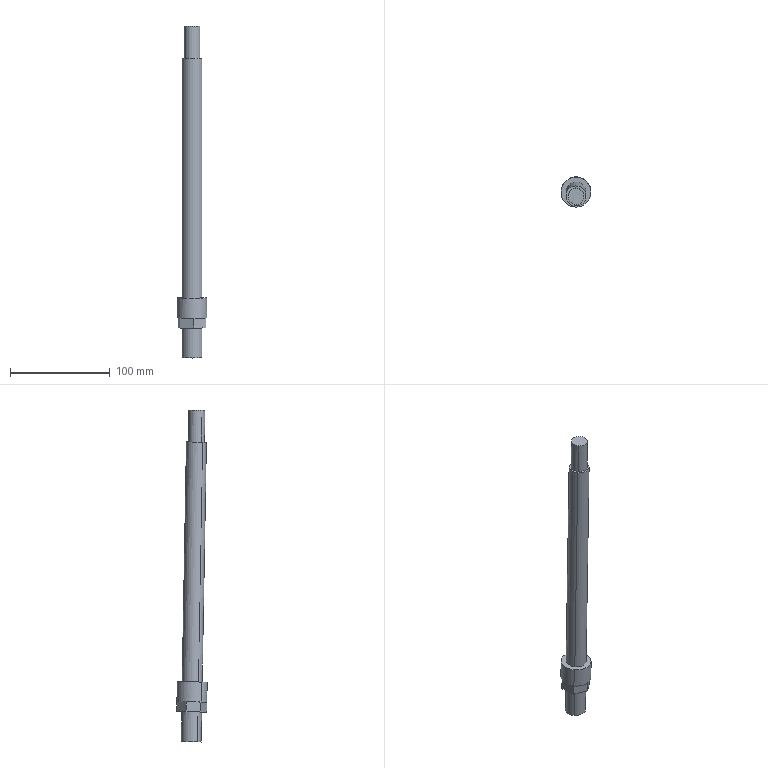Component | SolidWorks | SC63-50CylinderAxis-1 | 1 solid | 25 faces | box 30 x 30.39 x 332.26 mm | volume 111240 mm3 | plane 17 | cylinder 8 | commonest cylinder face diameters 20 x4 16 x2 30 x2
STEP:
#1=CARTESIAN_POINT('',(-1.02,48.421,1.561));
#2=VERTEX_POINT('',#1);
#3=CARTESIAN_POINT('',(-0.3966,48.901,1.569));
#4=VERTEX_POINT('',#3);
#5=CARTESIAN_POINT('',(-0.7085,48.661,1.565));
#6=DIRECTION('',(-0.,-0.01745,0.9998));
#7=DIRECTION('',(-0.7921,-0.6103,-0.01065));
#8=AXIS2_PLACEMENT_3D('',#5,#6,#7);
#9=CIRCLE('',#8,0.3937);
#10=EDGE_CURVE('',#2,#4,#9,.T.);
#11=ORIENTED_EDGE('',*,*,#10,.T.);
#12=CARTESIAN_POINT('',(-0.3966,48.881,2.75));
#13=VERTEX_POINT('',#12);
#14=CARTESIAN_POINT('',(-0.3966,48.673,14.638));
#15=DIRECTION('',(-0.,-0.01745,0.9998));
#16=VECTOR('',#15,39.37);
#17=LINE('',#14,#16);
#18=EDGE_CURVE('',#4,#13,#17,.T.);
#19=ORIENTED_EDGE('',*,*,#18,.T.);
#20=CARTESIAN_POINT('',(-1.02,48.4,2.742));
#21=VERTEX_POINT('',#20);
#22=CARTESIAN_POINT('',(-0.7085,48.641,2.746));
#23=DIRECTION('',(0.,0.01745,-0.9998));
#24=DIRECTION('',(0.7921,0.6103,0.01065));
#25=AXIS2_PLACEMENT_3D('',#22,#23,#24);
#26=CIRCLE('',#25,0.3937);
#27=EDGE_CURVE('',#13,#21,#26,.T.);
#28=ORIENTED_EDGE('',*,*,#27,.T.);
#29=CARTESIAN_POINT('',(-1.02,48.193,14.63));
#30=DIRECTION('',(-0.,-0.01745,0.9998));
#31=VECTOR('',#30,39.37);
#32=LINE('',#29,#31);
#33=EDGE_CURVE('',#2,#21,#32,.T.);
#34=ORIENTED_EDGE('',*,*,#33,.F.);
#35=EDGE_LOOP('',(#11,#19,#28,#34));
#36=FACE_OUTER_BOUND('',#35,.T.);
#37=CARTESIAN_POINT('',(-0.7085,48.433,14.634));
#38=DIRECTION('',(-0.,-0.01745,0.9998));
#39=DIRECTION('',(-0.7921,-0.6103,-0.01065));
#40=AXIS2_PLACEMENT_3D('',#37,#38,#39);
#41=CYLINDRICAL_SURFACE('',#40,0.3937);
#42=ADVANCED_FACE('',(#36),#41,.T.);
#43=CARTESIAN_POINT('',(-0.958,48.263,13.371));
#44=VERTEX_POINT('',#43);
#45=CARTESIAN_POINT('',(-0.459,48.647,13.378));
#46=VERTEX_POINT('',#45);
#47=CARTESIAN_POINT('',(-0.7085,48.455,13.374));
#48=DIRECTION('',(-0.,-0.01745,0.9998));
#49=DIRECTION('',(-0.7921,-0.6103,-0.01065));
#50=AXIS2_PLACEMENT_3D('',#47,#48,#49);
#51=CIRCLE('',#50,0.315);
#52=EDGE_CURVE('',#44,#46,#51,.T.);
#53=ORIENTED_EDGE('',*,*,#52,.T.);
#54=CARTESIAN_POINT('',(-0.459,48.625,14.637));
#55=VERTEX_POINT('',#54);
#56=CARTESIAN_POINT('',(-0.459,48.625,14.637));
#57=DIRECTION('',(-0.,-0.01745,0.9998));
#58=VECTOR('',#57,39.37);
#59=LINE('',#56,#58);
#60=EDGE_CURVE('',#46,#55,#59,.T.);
#61=ORIENTED_EDGE('',*,*,#60,.T.);
#62=CARTESIAN_POINT('',(-0.958,48.241,14.63));
#63=VERTEX_POINT('',#62);
#64=CARTESIAN_POINT('',(-0.7085,48.433,14.634));
#65=DIRECTION('',(-0.,-0.01745,0.9998));
#66=DIRECTION('',(-0.7921,-0.6103,-0.01065));
#67=AXIS2_PLACEMENT_3D('',#64,#65,#66);
#68=CIRCLE('',#67,0.315);
#69=EDGE_CURVE('',#63,#55,#68,.T.);
#70=ORIENTED_EDGE('',*,*,#69,.F.);
#71=CARTESIAN_POINT('',(-0.958,48.241,14.63));
#72=DIRECTION('',(-0.,-0.01745,0.9998));
#73=VECTOR('',#72,39.37);
#74=LINE('',#71,#73);
#75=EDGE_CURVE('',#44,#63,#74,.T.);
#76=ORIENTED_EDGE('',*,*,#75,.F.);
#77=EDGE_LOOP('',(#53,#61,#70,#76));
#78=FACE_OUTER_BOUND('',#77,.T.);
#79=CARTESIAN_POINT('',(-0.7085,48.433,14.634));
#80=DIRECTION('',(-0.,-0.01745,0.9998));
#81=DIRECTION('',(-0.7921,-0.6103,-0.01065));
#82=AXIS2_PLACEMENT_3D('',#79,#80,#81);
#83=CYLINDRICAL_SURFACE('',#82,0.315);
#84=ADVANCED_FACE('',(#78),#83,.T.);
#85=CARTESIAN_POINT('',(-0.3966,48.86,3.931));
#86=VERTEX_POINT('',#85);
#87=CARTESIAN_POINT('',(-1.02,48.38,3.923));
#88=VERTEX_POINT('',#87);
#89=CARTESIAN_POINT('',(-0.7085,48.62,3.927));
#90=DIRECTION('',(0.,0.01745,-0.9998));
#91=DIRECTION('',(0.7921,0.6103,0.01065));
#92=AXIS2_PLACEMENT_3D('',#89,#90,#91);
#93=CIRCLE('',#92,0.3937);
#94=EDGE_CURVE('',#86,#88,#93,.T.);
#95=ORIENTED_EDGE('',*,*,#94,.F.);
#96=CARTESIAN_POINT('',(-0.3966,48.695,13.378));
#97=VERTEX_POINT('',#96);
#98=CARTESIAN_POINT('',(-0.3966,48.673,14.638));
#99=DIRECTION('',(-0.,-0.01745,0.9998));
#100=VECTOR('',#99,39.37);
#101=LINE('',#98,#100);
#102=EDGE_CURVE('',#86,#97,#101,.T.);
#103=ORIENTED_EDGE('',*,*,#102,.T.);
#104=CARTESIAN_POINT('',(-1.02,48.215,13.37));
#105=VERTEX_POINT('',#104);
#106=CARTESIAN_POINT('',(-0.7085,48.455,13.374));
#107=DIRECTION('',(-0.,-0.01745,0.9998));
#108=DIRECTION('',(-0.7921,-0.6103,-0.01065));
#109=AXIS2_PLACEMENT_3D('',#106,#107,#108);
#110=CIRCLE('',#109,0.3937);
#111=EDGE_CURVE('',#105,#97,#110,.T.);
#112=ORIENTED_EDGE('',*,*,#111,.F.);
#113=CARTESIAN_POINT('',(-1.02,48.193,14.63));
#114=DIRECTION('',(-0.,-0.01745,0.9998));
#115=VECTOR('',#114,39.37);
#116=LINE('',#113,#115);
#117=EDGE_CURVE('',#88,#105,#116,.T.);
#118=ORIENTED_EDGE('',*,*,#117,.F.);
#119=EDGE_LOOP('',(#95,#103,#112,#118));
#120=FACE_OUTER_BOUND('',#119,.T.);
#121=CARTESIAN_POINT('',(-0.7085,48.433,14.634));
#122=DIRECTION('',(-0.,-0.01745,0.9998));
#123=DIRECTION('',(-0.7921,-0.6103,-0.01065));
#124=AXIS2_PLACEMENT_3D('',#121,#122,#123);
#125=CYLINDRICAL_SURFACE('',#124,0.3937);
#126=ADVANCED_FACE('',(#120),#125,.T.);
#127=CARTESIAN_POINT('',(-0.2407,48.98,3.933));
#128=VERTEX_POINT('',#127);
#129=CARTESIAN_POINT('',(-1.176,48.26,3.92));
#130=VERTEX_POINT('',#129);
#131=CARTESIAN_POINT('',(-0.7085,48.62,3.927));
#132=DIRECTION('',(0.,0.01745,-0.9998));
#133=DIRECTION('',(0.7921,0.6103,0.01065));
#134=AXIS2_PLACEMENT_3D('',#131,#132,#133);
#135=CIRCLE('',#134,0.5906);
#136=EDGE_CURVE('',#128,#130,#135,.T.);
#137=ORIENTED_EDGE('',*,*,#136,.T.);
#138=CARTESIAN_POINT('',(-1.176,48.273,3.133));
#139=VERTEX_POINT('',#138);
#140=CARTESIAN_POINT('',(-1.176,48.26,3.92));
#141=DIRECTION('',(0.,0.01745,-0.9998));
#142=VECTOR('',#141,39.37);
#143=LINE('',#140,#142);
#144=EDGE_CURVE('',#130,#139,#143,.T.);
#145=ORIENTED_EDGE('',*,*,#144,.T.);
#146=CARTESIAN_POINT('',(-0.6302,48.048,3.129));
#147=VERTEX_POINT('',#146);
#148=CARTESIAN_POINT('',(-0.7085,48.634,3.139));
#149=DIRECTION('',(-0.,-0.01745,0.9998));
#150=DIRECTION('',(0.7921,0.6103,0.01065));
#151=AXIS2_PLACEMENT_3D('',#148,#149,#150);
#152=CIRCLE('',#151,0.5906);
#153=EDGE_CURVE('',#139,#147,#152,.T.);
#154=ORIENTED_EDGE('',*,*,#153,.T.);
#155=CARTESIAN_POINT('',(-0.1625,48.409,3.136));
#156=VERTEX_POINT('',#155);
#157=CARTESIAN_POINT('',(-0.7085,48.634,3.139));
#158=DIRECTION('',(-0.,-0.01745,0.9998));
#159=DIRECTION('',(0.7921,0.6103,0.01065));
#160=AXIS2_PLACEMENT_3D('',#157,#158,#159);
#161=CIRCLE('',#160,0.5906);
#162=EDGE_CURVE('',#147,#156,#161,.T.);
#163=ORIENTED_EDGE('',*,*,#162,.T.);
#164=CARTESIAN_POINT('',(-0.2407,48.994,3.146));
#165=VERTEX_POINT('',#164);
#166=CARTESIAN_POINT('',(-0.7085,48.634,3.139));
#167=DIRECTION('',(-0.,-0.01745,0.9998));
#168=DIRECTION('',(0.7921,0.6103,0.01065));
#169=AXIS2_PLACEMENT_3D('',#166,#167,#168);
#170=CIRCLE('',#169,0.5906);
#171=EDGE_CURVE('',#156,#165,#170,.T.);
#172=ORIENTED_EDGE('',*,*,#171,.T.);
#173=CARTESIAN_POINT('',(-0.2407,48.98,3.933));
#174=DIRECTION('',(0.,0.01745,-0.9998));
#175=VECTOR('',#174,39.37);
#176=LINE('',#173,#175);
#177=EDGE_CURVE('',#128,#165,#176,.T.);
#178=ORIENTED_EDGE('',*,*,#177,.F.);
#179=EDGE_LOOP('',(#137,#145,#154,#163,#172,#178));
#180=FACE_OUTER_BOUND('',#179,.T.);
#181=CARTESIAN_POINT('',(-0.7085,48.62,3.927));
#182=DIRECTION('',(0.,0.01745,-0.9998));
#183=DIRECTION('',(0.7921,0.6103,0.01065));
#184=AXIS2_PLACEMENT_3D('',#181,#182,#183);
#185=CYLINDRICAL_SURFACE('',#184,0.5906);
#186=ADVANCED_FACE('',(#180),#185,.T.);
#187=ORIENTED_EDGE('',*,*,#144,.F.);
#188=CARTESIAN_POINT('',(-0.7085,48.62,3.927));
#189=DIRECTION('',(0.,0.01745,-0.9998));
#190=DIRECTION('',(0.7921,0.6103,0.01065));
#191=AXIS2_PLACEMENT_3D('',#188,#189,#190);
#192=CIRCLE('',#191,0.5906);
#193=EDGE_CURVE('',#130,#128,#192,.T.);
#194=ORIENTED_EDGE('',*,*,#193,.T.);
#195=ORIENTED_EDGE('',*,*,#177,.T.);
#196=CARTESIAN_POINT('',(-0.7868,49.219,3.15));
#197=VERTEX_POINT('',#196);
#198=CARTESIAN_POINT('',(-0.7085,48.634,3.139));
#199=DIRECTION('',(-0.,-0.01745,0.9998));
#200=DIRECTION('',(0.7921,0.6103,0.01065));
#201=AXIS2_PLACEMENT_3D('',#198,#199,#200);
#202=CIRCLE('',#201,0.5906);
#203=EDGE_CURVE('',#165,#197,#202,.T.);
#204=ORIENTED_EDGE('',*,*,#203,.T.);
#205=CARTESIAN_POINT('',(-1.255,48.859,3.143));
#206=VERTEX_POINT('',#205);
#207=CARTESIAN_POINT('',(-0.7085,48.634,3.139));
#208=DIRECTION('',(-0.,-0.01745,0.9998));
#209=DIRECTION('',(0.7921,0.6103,0.01065));
#210=AXIS2_PLACEMENT_3D('',#207,#208,#209);
#211=CIRCLE('',#210,0.5906);
#212=EDGE_CURVE('',#197,#206,#211,.T.);
#213=ORIENTED_EDGE('',*,*,#212,.T.);
#214=CARTESIAN_POINT('',(-0.7085,48.634,3.139));
#215=DIRECTION('',(-0.,-0.01745,0.9998));
#216=DIRECTION('',(0.7921,0.6103,0.01065));
#217=AXIS2_PLACEMENT_3D('',#214,#215,#216);
#218=CIRCLE('',#217,0.5906);
#219=EDGE_CURVE('',#206,#139,#218,.T.);
#220=ORIENTED_EDGE('',*,*,#219,.T.);
#221=EDGE_LOOP('',(#187,#194,#195,#204,#213,#220));
#222=FACE_OUTER_BOUND('',#221,.T.);
#223=CARTESIAN_POINT('',(-0.7085,48.62,3.927));
#224=DIRECTION('',(0.,0.01745,-0.9998));
#225=DIRECTION('',(0.7921,0.6103,0.01065));
#226=AXIS2_PLACEMENT_3D('',#223,#224,#225);
#227=CYLINDRICAL_SURFACE('',#226,0.5906);
#228=ADVANCED_FACE('',(#222),#227,.T.);
#229=ORIENTED_EDGE('',*,*,#102,.F.);
#230=CARTESIAN_POINT('',(-0.7085,48.62,3.927));
#231=DIRECTION('',(0.,0.01745,-0.9998));
#232=DIRECTION('',(0.7921,0.6103,0.01065));
#233=AXIS2_PLACEMENT_3D('',#230,#231,#232);
#234=CIRCLE('',#233,0.3937);
#235=EDGE_CURVE('',#88,#86,#234,.T.);
#236=ORIENTED_EDGE('',*,*,#235,.F.);
#237=ORIENTED_EDGE('',*,*,#117,.T.);
#238=CARTESIAN_POINT('',(-0.7085,48.455,13.374));
#239=DIRECTION('',(-0.,-0.01745,0.9998));
#240=DIRECTION('',(-0.7921,-0.6103,-0.01065));
#241=AXIS2_PLACEMENT_3D('',#238,#239,#240);
#242=CIRCLE('',#241,0.3937);
#243=EDGE_CURVE('',#97,#105,#242,.T.);
#244=ORIENTED_EDGE('',*,*,#243,.F.);
#245=EDGE_LOOP('',(#229,#236,#237,#244));
#246=FACE_OUTER_BOUND('',#245,.T.);
#247=CARTESIAN_POINT('',(-0.7085,48.433,14.634));
#248=DIRECTION('',(-0.,-0.01745,0.9998));
#249=DIRECTION('',(-0.7921,-0.6103,-0.01065));
#250=AXIS2_PLACEMENT_3D('',#247,#248,#249);
#251=CYLINDRICAL_SURFACE('',#250,0.3937);
#252=ADVANCED_FACE('',(#246),#251,.T.);
#253=ORIENTED_EDGE('',*,*,#69,.T.);
#254=CARTESIAN_POINT('',(-0.7085,48.433,14.634));
#255=DIRECTION('',(-0.,-0.01745,0.9998));
#256=DIRECTION('',(-0.7921,-0.6103,-0.01065));
#257=AXIS2_PLACEMENT_3D('',#254,#255,#256);
#258=CIRCLE('',#257,0.315);
#259=EDGE_CURVE('',#55,#63,#258,.T.);
#260=ORIENTED_EDGE('',*,*,#259,.T.);
#261=EDGE_LOOP('',(#253,#260));
#262=FACE_OUTER_BOUND('',#261,.T.);
#263=CARTESIAN_POINT('',(-0.7085,48.433,14.634));
#264=DIRECTION('',(0.,0.01745,-0.9998));
#265=DIRECTION('',(0.7921,0.6103,0.01065));
#266=AXIS2_PLACEMENT_3D('',#263,#264,#265);
#267=PLANE('',#266);
#268=ADVANCED_FACE('',(#262),#267,.F.);
#269=ORIENTED_EDGE('',*,*,#60,.F.);
#270=CARTESIAN_POINT('',(-0.7085,48.455,13.374));
#271=DIRECTION('',(-0.,-0.01745,0.9998));
#272=DIRECTION('',(-0.7921,-0.6103,-0.01065));
#273=AXIS2_PLACEMENT_3D('',#270,#271,#272);
#274=CIRCLE('',#273,0.315);
#275=EDGE_CURVE('',#46,#44,#274,.T.);
#276=ORIENTED_EDGE('',*,*,#275,.T.);
#277=ORIENTED_EDGE('',*,*,#75,.T.);
#278=ORIENTED_EDGE('',*,*,#259,.F.);
#279=EDGE_LOOP('',(#269,#276,#277,#278));
#280=FACE_OUTER_BOUND('',#279,.T.);
#281=CARTESIAN_POINT('',(-0.7085,48.433,14.634));
#282=DIRECTION('',(-0.,-0.01745,0.9998));
#283=DIRECTION('',(-0.7921,-0.6103,-0.01065));
#284=AXIS2_PLACEMENT_3D('',#281,#282,#283);
#285=CYLINDRICAL_SURFACE('',#284,0.315);
#286=ADVANCED_FACE('',(#280),#285,.T.);
#287=ORIENTED_EDGE('',*,*,#52,.F.);
#288=ORIENTED_EDGE('',*,*,#275,.F.);
#289=EDGE_LOOP('',(#287,#288));
#290=FACE_BOUND('',#289,.T.);
#291=ORIENTED_EDGE('',*,*,#111,.T.);
#292=ORIENTED_EDGE('',*,*,#243,.T.);
#293=EDGE_LOOP('',(#291,#292));
#294=FACE_OUTER_BOUND('',#293,.T.);
#295=CARTESIAN_POINT('',(-0.5163,48.206,13.37));
#296=DIRECTION('',(0.,0.01745,-0.9998));
#297=DIRECTION('',(0.7921,0.6103,0.01065));
#298=AXIS2_PLACEMENT_3D('',#295,#296,#297);
#299=PLANE('',#298);
#300=ADVANCED_FACE('',(#290,#294),#299,.F.);
#301=ORIENTED_EDGE('',*,*,#235,.T.);
#302=ORIENTED_EDGE('',*,*,#94,.T.);
#303=EDGE_LOOP('',(#301,#302));
#304=FACE_BOUND('',#303,.T.);
#305=ORIENTED_EDGE('',*,*,#136,.F.);
#306=ORIENTED_EDGE('',*,*,#193,.F.);
#307=EDGE_LOOP('',(#305,#306));
#308=FACE_OUTER_BOUND('',#307,.T.);
#309=CARTESIAN_POINT('',(-0.7085,48.62,3.927));
#310=DIRECTION('',(0.,0.01745,-0.9998));
#311=DIRECTION('',(0.7921,0.6103,0.01065));
#312=AXIS2_PLACEMENT_3D('',#309,#310,#311);
#313=PLANE('',#312);
#314=ADVANCED_FACE('',(#304,#308),#313,.F.);
#315=CARTESIAN_POINT('',(-0.7868,49.219,3.15));
#316=DIRECTION('',(0.9246,-0.3808,-0.006646));
#317=VECTOR('',#316,39.37);
#318=LINE('',#315,#317);
#319=EDGE_CURVE('',#197,#165,#318,.T.);
#320=ORIENTED_EDGE('',*,*,#319,.F.);
#321=ORIENTED_EDGE('',*,*,#203,.F.);
#322=EDGE_LOOP('',(#320,#321));
#323=FACE_OUTER_BOUND('',#322,.T.);
#324=CARTESIAN_POINT('',(-0.7085,48.634,3.139));
#325=DIRECTION('',(0.,0.01745,-0.9998));
#326=DIRECTION('',(0.7921,0.6103,0.01065));
#327=AXIS2_PLACEMENT_3D('',#324,#325,#326);
#328=PLANE('',#327);
#329=ADVANCED_FACE('',(#323),#328,.T.);
#330=CARTESIAN_POINT('',(-1.255,48.859,3.143));
#331=DIRECTION('',(0.7921,0.6103,0.01065));
#332=VECTOR('',#331,39.37);
#333=LINE('',#330,#332);
#334=EDGE_CURVE('',#206,#197,#333,.T.);
#335=ORIENTED_EDGE('',*,*,#334,.F.);
#336=ORIENTED_EDGE('',*,*,#212,.F.);
#337=EDGE_LOOP('',(#335,#336));
#338=FACE_OUTER_BOUND('',#337,.T.);
#339=CARTESIAN_POINT('',(-0.7085,48.634,3.139));
#340=DIRECTION('',(0.,0.01745,-0.9998));
#341=DIRECTION('',(0.7921,0.6103,0.01065));
#342=AXIS2_PLACEMENT_3D('',#339,#340,#341);
#343=PLANE('',#342);
#344=ADVANCED_FACE('',(#338),#343,.T.);
#345=CARTESIAN_POINT('',(-1.176,48.273,3.133));
#346=DIRECTION('',(-0.1325,0.991,0.0173));
#347=VECTOR('',#346,39.37);
#348=LINE('',#345,#347);
#349=EDGE_CURVE('',#139,#206,#348,.T.);
#350=ORIENTED_EDGE('',*,*,#349,.F.);
#351=ORIENTED_EDGE('',*,*,#219,.F.);
#352=EDGE_LOOP('',(#350,#351));
#353=FACE_OUTER_BOUND('',#352,.T.);
#354=CARTESIAN_POINT('',(-0.7085,48.634,3.139));
#355=DIRECTION('',(0.,0.01745,-0.9998));
#356=DIRECTION('',(0.7921,0.6103,0.01065));
#357=AXIS2_PLACEMENT_3D('',#354,#355,#356);
#358=PLANE('',#357);
#359=ADVANCED_FACE('',(#353),#358,.T.);
#360=CARTESIAN_POINT('',(-0.6302,48.048,3.129));
#361=DIRECTION('',(-0.9246,0.3808,0.006646));
#362=VECTOR('',#361,39.37);
#363=LINE('',#360,#362);
#364=EDGE_CURVE('',#147,#139,#363,.T.);
#365=ORIENTED_EDGE('',*,*,#364,.F.);
#366=ORIENTED_EDGE('',*,*,#153,.F.);
#367=EDGE_LOOP('',(#365,#366));
#368=FACE_OUTER_BOUND('',#367,.T.);
#369=CARTESIAN_POINT('',(-0.7085,48.634,3.139));
#370=DIRECTION('',(0.,0.01745,-0.9998));
#371=DIRECTION('',(0.7921,0.6103,0.01065));
#372=AXIS2_PLACEMENT_3D('',#369,#370,#371);
#373=PLANE('',#372);
#374=ADVANCED_FACE('',(#368),#373,.T.);
#375=CARTESIAN_POINT('',(-0.1625,48.409,3.136));
#376=DIRECTION('',(-0.7921,-0.6103,-0.01065));
#377=VECTOR('',#376,39.37);
#378=LINE('',#375,#377);
#379=EDGE_CURVE('',#156,#147,#378,.T.);
#380=ORIENTED_EDGE('',*,*,#379,.F.);
#381=ORIENTED_EDGE('',*,*,#162,.F.);
#382=EDGE_LOOP('',(#380,#381));
#383=FACE_OUTER_BOUND('',#382,.T.);
#384=CARTESIAN_POINT('',(-0.7085,48.634,3.139));
#385=DIRECTION('',(0.,0.01745,-0.9998));
#386=DIRECTION('',(0.7921,0.6103,0.01065));
#387=AXIS2_PLACEMENT_3D('',#384,#385,#386);
#388=PLANE('',#387);
#389=ADVANCED_FACE('',(#383),#388,.T.);
#390=CARTESIAN_POINT('',(-0.2407,48.994,3.146));
#391=DIRECTION('',(0.1325,-0.991,-0.0173));
#392=VECTOR('',#391,39.37);
#393=LINE('',#390,#392);
#394=EDGE_CURVE('',#165,#156,#393,.T.);
#395=ORIENTED_EDGE('',*,*,#394,.F.);
#396=ORIENTED_EDGE('',*,*,#171,.F.);
#397=EDGE_LOOP('',(#395,#396));
#398=FACE_OUTER_BOUND('',#397,.T.);
#399=CARTESIAN_POINT('',(-0.7085,48.634,3.139));
#400=DIRECTION('',(0.,0.01745,-0.9998));
#401=DIRECTION('',(0.7921,0.6103,0.01065));
#402=AXIS2_PLACEMENT_3D('',#399,#400,#401);
#403=PLANE('',#402);
#404=ADVANCED_FACE('',(#398),#403,.T.);
#405=CARTESIAN_POINT('',(-0.7868,49.226,2.756));
#406=VERTEX_POINT('',#405);
#407=CARTESIAN_POINT('',(-0.2407,49.001,2.752));
#408=VERTEX_POINT('',#407);
#409=CARTESIAN_POINT('',(-0.7868,49.226,2.756));
#410=DIRECTION('',(0.9246,-0.3808,-0.006646));
#411=VECTOR('',#410,39.37);
#412=LINE('',#409,#411);
#413=EDGE_CURVE('',#406,#408,#412,.T.);
#414=ORIENTED_EDGE('',*,*,#413,.F.);
#415=CARTESIAN_POINT('',(-0.7868,49.219,3.15));
#416=DIRECTION('',(0.,0.01745,-0.9998));
#417=VECTOR('',#416,39.37);
#418=LINE('',#415,#417);
#419=EDGE_CURVE('',#197,#406,#418,.T.);
#420=ORIENTED_EDGE('',*,*,#419,.F.);
#421=ORIENTED_EDGE('',*,*,#319,.T.);
#422=CARTESIAN_POINT('',(-0.2407,48.994,3.146));
#423=DIRECTION('',(0.,0.01745,-0.9998));
#424=VECTOR('',#423,39.37);
#425=LINE('',#422,#424);
#426=EDGE_CURVE('',#165,#408,#425,.T.);
#427=ORIENTED_EDGE('',*,*,#426,.T.);
#428=EDGE_LOOP('',(#414,#420,#421,#427));
#429=FACE_OUTER_BOUND('',#428,.T.);
#430=CARTESIAN_POINT('',(-0.7868,49.219,3.15));
#431=DIRECTION('',(0.3808,0.9245,0.01614));
#432=DIRECTION('',(0.9246,-0.3808,-0.006646));
#433=AXIS2_PLACEMENT_3D('',#430,#431,#432);
#434=PLANE('',#433);
#435=ADVANCED_FACE('',(#429),#434,.T.);
#436=CARTESIAN_POINT('',(-1.255,48.865,2.75));
#437=VERTEX_POINT('',#436);
#438=CARTESIAN_POINT('',(-1.255,48.865,2.75));
#439=DIRECTION('',(0.7921,0.6103,0.01065));
#440=VECTOR('',#439,39.37);
#441=LINE('',#438,#440);
#442=EDGE_CURVE('',#437,#406,#441,.T.);
#443=ORIENTED_EDGE('',*,*,#442,.F.);
#444=CARTESIAN_POINT('',(-1.255,48.859,3.143));
#445=DIRECTION('',(0.,0.01745,-0.9998));
#446=VECTOR('',#445,39.37);
#447=LINE('',#444,#446);
#448=EDGE_CURVE('',#206,#437,#447,.T.);
#449=ORIENTED_EDGE('',*,*,#448,.F.);
#450=ORIENTED_EDGE('',*,*,#334,.T.);
#451=ORIENTED_EDGE('',*,*,#419,.T.);
#452=EDGE_LOOP('',(#443,#449,#450,#451));
#453=FACE_OUTER_BOUND('',#452,.T.);
#454=CARTESIAN_POINT('',(-1.255,48.859,3.143));
#455=DIRECTION('',(-0.6104,0.792,0.01382));
#456=DIRECTION('',(0.7921,0.6103,0.01065));
#457=AXIS2_PLACEMENT_3D('',#454,#455,#456);
#458=PLANE('',#457);
#459=ADVANCED_FACE('',(#453),#458,.T.);
#460=CARTESIAN_POINT('',(-1.176,48.28,2.74));
#461=VERTEX_POINT('',#460);
#462=CARTESIAN_POINT('',(-1.176,48.28,2.74));
#463=DIRECTION('',(-0.1325,0.991,0.0173));
#464=VECTOR('',#463,39.37);
#465=LINE('',#462,#464);
#466=EDGE_CURVE('',#461,#437,#465,.T.);
#467=ORIENTED_EDGE('',*,*,#466,.F.);
#468=CARTESIAN_POINT('',(-1.176,48.273,3.133));
#469=DIRECTION('',(0.,0.01745,-0.9998));
#470=VECTOR('',#469,39.37);
#471=LINE('',#468,#470);
#472=EDGE_CURVE('',#139,#461,#471,.T.);
#473=ORIENTED_EDGE('',*,*,#472,.F.);
#474=ORIENTED_EDGE('',*,*,#349,.T.);
#475=ORIENTED_EDGE('',*,*,#448,.T.);
#476=EDGE_LOOP('',(#467,#473,#474,#475));
#477=FACE_OUTER_BOUND('',#476,.T.);
#478=CARTESIAN_POINT('',(-1.176,48.273,3.133));
#479=DIRECTION('',(-0.9912,-0.1325,-0.002313));
#480=DIRECTION('',(-0.1325,0.991,0.0173));
#481=AXIS2_PLACEMENT_3D('',#478,#479,#480);
#482=PLANE('',#481);
#483=ADVANCED_FACE('',(#477),#482,.T.);
#484=CARTESIAN_POINT('',(-0.6302,48.055,2.736));
#485=VERTEX_POINT('',#484);
#486=CARTESIAN_POINT('',(-0.6302,48.055,2.736));
#487=DIRECTION('',(-0.9246,0.3808,0.006646));
#488=VECTOR('',#487,39.37);
#489=LINE('',#486,#488);
#490=EDGE_CURVE('',#485,#461,#489,.T.);
#491=ORIENTED_EDGE('',*,*,#490,.F.);
#492=CARTESIAN_POINT('',(-0.6302,48.048,3.129));
#493=DIRECTION('',(0.,0.01745,-0.9998));
#494=VECTOR('',#493,39.37);
#495=LINE('',#492,#494);
#496=EDGE_CURVE('',#147,#485,#495,.T.);
#497=ORIENTED_EDGE('',*,*,#496,.F.);
#498=ORIENTED_EDGE('',*,*,#364,.T.);
#499=ORIENTED_EDGE('',*,*,#472,.T.);
#500=EDGE_LOOP('',(#491,#497,#498,#499));
#501=FACE_OUTER_BOUND('',#500,.T.);
#502=CARTESIAN_POINT('',(-0.6302,48.048,3.129));
#503=DIRECTION('',(-0.3808,-0.9245,-0.01614));
#504=DIRECTION('',(-0.9246,0.3808,0.006646));
#505=AXIS2_PLACEMENT_3D('',#502,#503,#504);
#506=PLANE('',#505);
#507=ADVANCED_FACE('',(#501),#506,.T.);
#508=CARTESIAN_POINT('',(-0.1625,48.416,2.742));
#509=VERTEX_POINT('',#508);
#510=CARTESIAN_POINT('',(-0.1625,48.416,2.742));
#511=DIRECTION('',(-0.7921,-0.6103,-0.01065));
#512=VECTOR('',#511,39.37);
#513=LINE('',#510,#512);
#514=EDGE_CURVE('',#509,#485,#513,.T.);
#515=ORIENTED_EDGE('',*,*,#514,.F.);
#516=CARTESIAN_POINT('',(-0.1625,48.409,3.136));
#517=DIRECTION('',(0.,0.01745,-0.9998));
#518=VECTOR('',#517,39.37);
#519=LINE('',#516,#518);
#520=EDGE_CURVE('',#156,#509,#519,.T.);
#521=ORIENTED_EDGE('',*,*,#520,.F.);
#522=ORIENTED_EDGE('',*,*,#379,.T.);
#523=ORIENTED_EDGE('',*,*,#496,.T.);
#524=EDGE_LOOP('',(#515,#521,#522,#523));
#525=FACE_OUTER_BOUND('',#524,.T.);
#526=CARTESIAN_POINT('',(-0.1625,48.409,3.136));
#527=DIRECTION('',(0.6104,-0.792,-0.01382));
#528=DIRECTION('',(-0.7921,-0.6103,-0.01065));
#529=AXIS2_PLACEMENT_3D('',#526,#527,#528);
#530=PLANE('',#529);
#531=ADVANCED_FACE('',(#525),#530,.T.);
#532=CARTESIAN_POINT('',(-0.2407,49.001,2.752));
#533=DIRECTION('',(0.1325,-0.991,-0.0173));
#534=VECTOR('',#533,39.37);
#535=LINE('',#532,#534);
#536=EDGE_CURVE('',#408,#509,#535,.T.);
#537=ORIENTED_EDGE('',*,*,#536,.F.);
#538=ORIENTED_EDGE('',*,*,#426,.F.);
#539=ORIENTED_EDGE('',*,*,#394,.T.);
#540=ORIENTED_EDGE('',*,*,#520,.T.);
#541=EDGE_LOOP('',(#537,#538,#539,#540));
#542=FACE_OUTER_BOUND('',#541,.T.);
#543=CARTESIAN_POINT('',(-0.2407,48.994,3.146));
#544=DIRECTION('',(0.9912,0.1325,0.002313));
#545=DIRECTION('',(0.1325,-0.991,-0.0173));
#546=AXIS2_PLACEMENT_3D('',#543,#544,#545);
#547=PLANE('',#546);
#548=ADVANCED_FACE('',(#542),#547,.T.);
#549=ORIENTED_EDGE('',*,*,#10,.F.);
#550=CARTESIAN_POINT('',(-0.7085,48.661,1.565));
#551=DIRECTION('',(-0.,-0.01745,0.9998));
#552=DIRECTION('',(-0.7921,-0.6103,-0.01065));
#553=AXIS2_PLACEMENT_3D('',#550,#551,#552);
#554=CIRCLE('',#553,0.3937);
#555=EDGE_CURVE('',#4,#2,#554,.T.);
#556=ORIENTED_EDGE('',*,*,#555,.F.);
#557=EDGE_LOOP('',(#549,#556));
#558=FACE_OUTER_BOUND('',#557,.T.);
#559=CARTESIAN_POINT('',(-0.4682,48.349,1.559));
#560=DIRECTION('',(-0.,-0.01745,0.9998));
#561=DIRECTION('',(-0.7921,-0.6103,-0.01065));
#562=AXIS2_PLACEMENT_3D('',#559,#560,#561);
#563=PLANE('',#562);
#564=ADVANCED_FACE('',(#558),#563,.F.);
#565=ORIENTED_EDGE('',*,*,#18,.F.);
#566=ORIENTED_EDGE('',*,*,#555,.T.);
#567=ORIENTED_EDGE('',*,*,#33,.T.);
#568=CARTESIAN_POINT('',(-0.7085,48.641,2.746));
#569=DIRECTION('',(0.,0.01745,-0.9998));
#570=DIRECTION('',(0.7921,0.6103,0.01065));
#571=AXIS2_PLACEMENT_3D('',#568,#569,#570);
#572=CIRCLE('',#571,0.3937);
#573=EDGE_CURVE('',#21,#13,#572,.T.);
#574=ORIENTED_EDGE('',*,*,#573,.T.);
#575=EDGE_LOOP('',(#565,#566,#567,#574));
#576=FACE_OUTER_BOUND('',#575,.T.);
#577=CARTESIAN_POINT('',(-0.7085,48.433,14.634));
#578=DIRECTION('',(-0.,-0.01745,0.9998));
#579=DIRECTION('',(-0.7921,-0.6103,-0.01065));
#580=AXIS2_PLACEMENT_3D('',#577,#578,#579);
#581=CYLINDRICAL_SURFACE('',#580,0.3937);
#582=ADVANCED_FACE('',(#576),#581,.T.);
#583=ORIENTED_EDGE('',*,*,#573,.F.);
#584=ORIENTED_EDGE('',*,*,#27,.F.);
#585=EDGE_LOOP('',(#583,#584));
#586=FACE_BOUND('',#585,.T.);
#587=ORIENTED_EDGE('',*,*,#442,.T.);
#588=ORIENTED_EDGE('',*,*,#413,.T.);
#589=ORIENTED_EDGE('',*,*,#536,.T.);
#590=ORIENTED_EDGE('',*,*,#514,.T.);
#591=ORIENTED_EDGE('',*,*,#490,.T.);
#592=ORIENTED_EDGE('',*,*,#466,.T.);
#593=EDGE_LOOP('',(#587,#588,#589,#590,#591,#592));
#594=FACE_OUTER_BOUND('',#593,.T.);
#595=CARTESIAN_POINT('',(-0.7085,48.641,2.746));
#596=DIRECTION('',(0.,0.01745,-0.9998));
#597=DIRECTION('',(0.7921,0.6103,0.01065));
#598=AXIS2_PLACEMENT_3D('',#595,#596,#597);
#599=PLANE('',#598);
#600=ADVANCED_FACE('',(#586,#594),#599,.T.);
#601=CLOSED_SHELL('',(#42,#84,#126,#186,#228,#252,#268,#286,#300,#314,#329,#344,#359,#374,#389,#404,#435,#459,#483,#507,#531,#548,#564,#582,#600));
#602=MANIFOLD_SOLID_BREP('',#601);
#603=CARTESIAN_POINT('',(0.,0.,0.));
#604=DIRECTION('',(0.,0.,1.));
#605=DIRECTION('',(1.,0.,0.));
#606=AXIS2_PLACEMENT_3D('',#603,#604,#605);
#607=(LENGTH_UNIT()NAMED_UNIT(*)SI_UNIT($,.METRE.));
#608=LENGTH_MEASURE_WITH_UNIT(LENGTH_MEASURE(0.0254),#607);
#609=DIMENSIONAL_EXPONENTS(1.,0.,0.,0.,0.,0.,0.);
#610=(CONVERSION_BASED_UNIT('',#608)LENGTH_UNIT()NAMED_UNIT(#609));
#611=UNCERTAINTY_MEASURE_WITH_UNIT(LENGTH_MEASURE(0.00001),#610,'','');
#612=(NAMED_UNIT(*)PLANE_ANGLE_UNIT()SI_UNIT($,.RADIAN.));
#613=(NAMED_UNIT(*)SI_UNIT($,.STERADIAN.)SOLID_ANGLE_UNIT());
#614=(GEOMETRIC_REPRESENTATION_CONTEXT(3)GLOBAL_UNCERTAINTY_ASSIGNED_CONTEXT((#611))GLOBAL_UNIT_ASSIGNED_CONTEXT((#610,#612,#613))REPRESENTATION_CONTEXT('',''));
#615=ADVANCED_BREP_SHAPE_REPRESENTATION('',(#602,#606),#614);
#616=COLOUR_RGB('',0.7922,0.8196,0.9333);
#617=FILL_AREA_STYLE_COLOUR('',#616);
#618=FILL_AREA_STYLE('',(#617));
#619=SURFACE_STYLE_FILL_AREA(#618);
#620=SURFACE_SIDE_STYLE('',(#619));
#621=SURFACE_STYLE_USAGE(.BOTH.,#620);
#622=PRESENTATION_STYLE_ASSIGNMENT((#621));
#623=STYLED_ITEM('',(#622),#602);
#624=PRESENTATION_LAYER_ASSIGNMENT('','',(#623));
#625=(LENGTH_UNIT()NAMED_UNIT(*)SI_UNIT($,.METRE.));
#626=LENGTH_MEASURE_WITH_UNIT(LENGTH_MEASURE(0.0254),#625);
#627=DIMENSIONAL_EXPONENTS(1.,0.,0.,0.,0.,0.,0.);
#628=(CONVERSION_BASED_UNIT('',#626)LENGTH_UNIT()NAMED_UNIT(#627));
#629=UNCERTAINTY_MEASURE_WITH_UNIT(LENGTH_MEASURE(0.00001),#628,'','');
#630=(NAMED_UNIT(*)PLANE_ANGLE_UNIT()SI_UNIT($,.RADIAN.));
#631=(NAMED_UNIT(*)SI_UNIT($,.STERADIAN.)SOLID_ANGLE_UNIT());
#632=(GEOMETRIC_REPRESENTATION_CONTEXT(3)GLOBAL_UNCERTAINTY_ASSIGNED_CONTEXT((#629))GLOBAL_UNIT_ASSIGNED_CONTEXT((#628,#630,#631))REPRESENTATION_CONTEXT('',''));
#633=MECHANICAL_DESIGN_GEOMETRIC_PRESENTATION_REPRESENTATION('',(#623),#632);